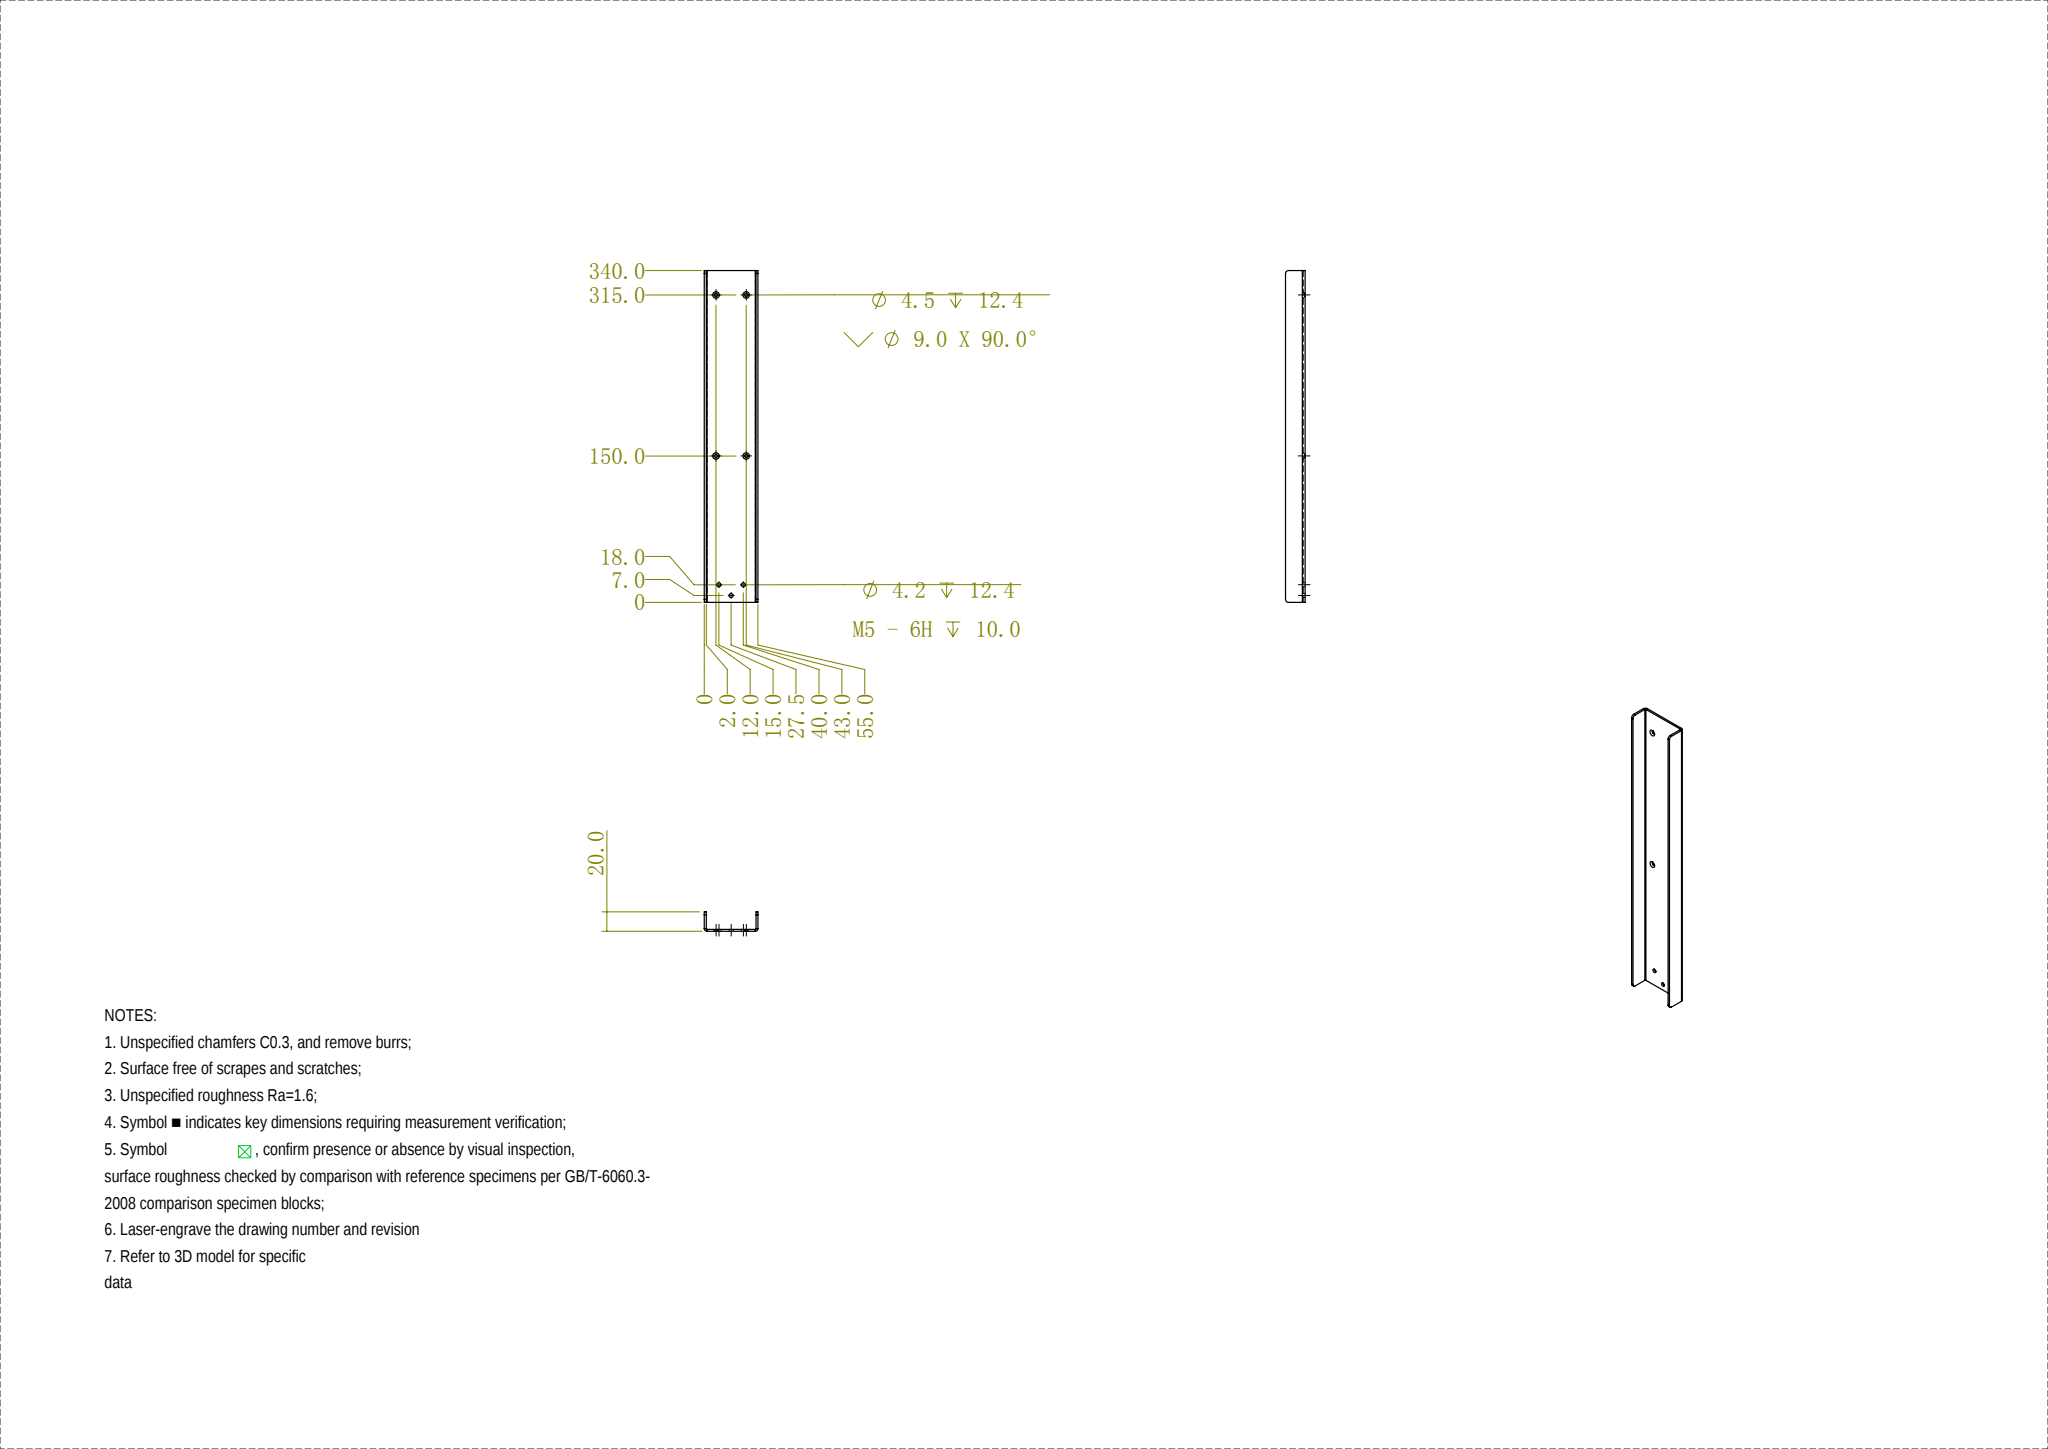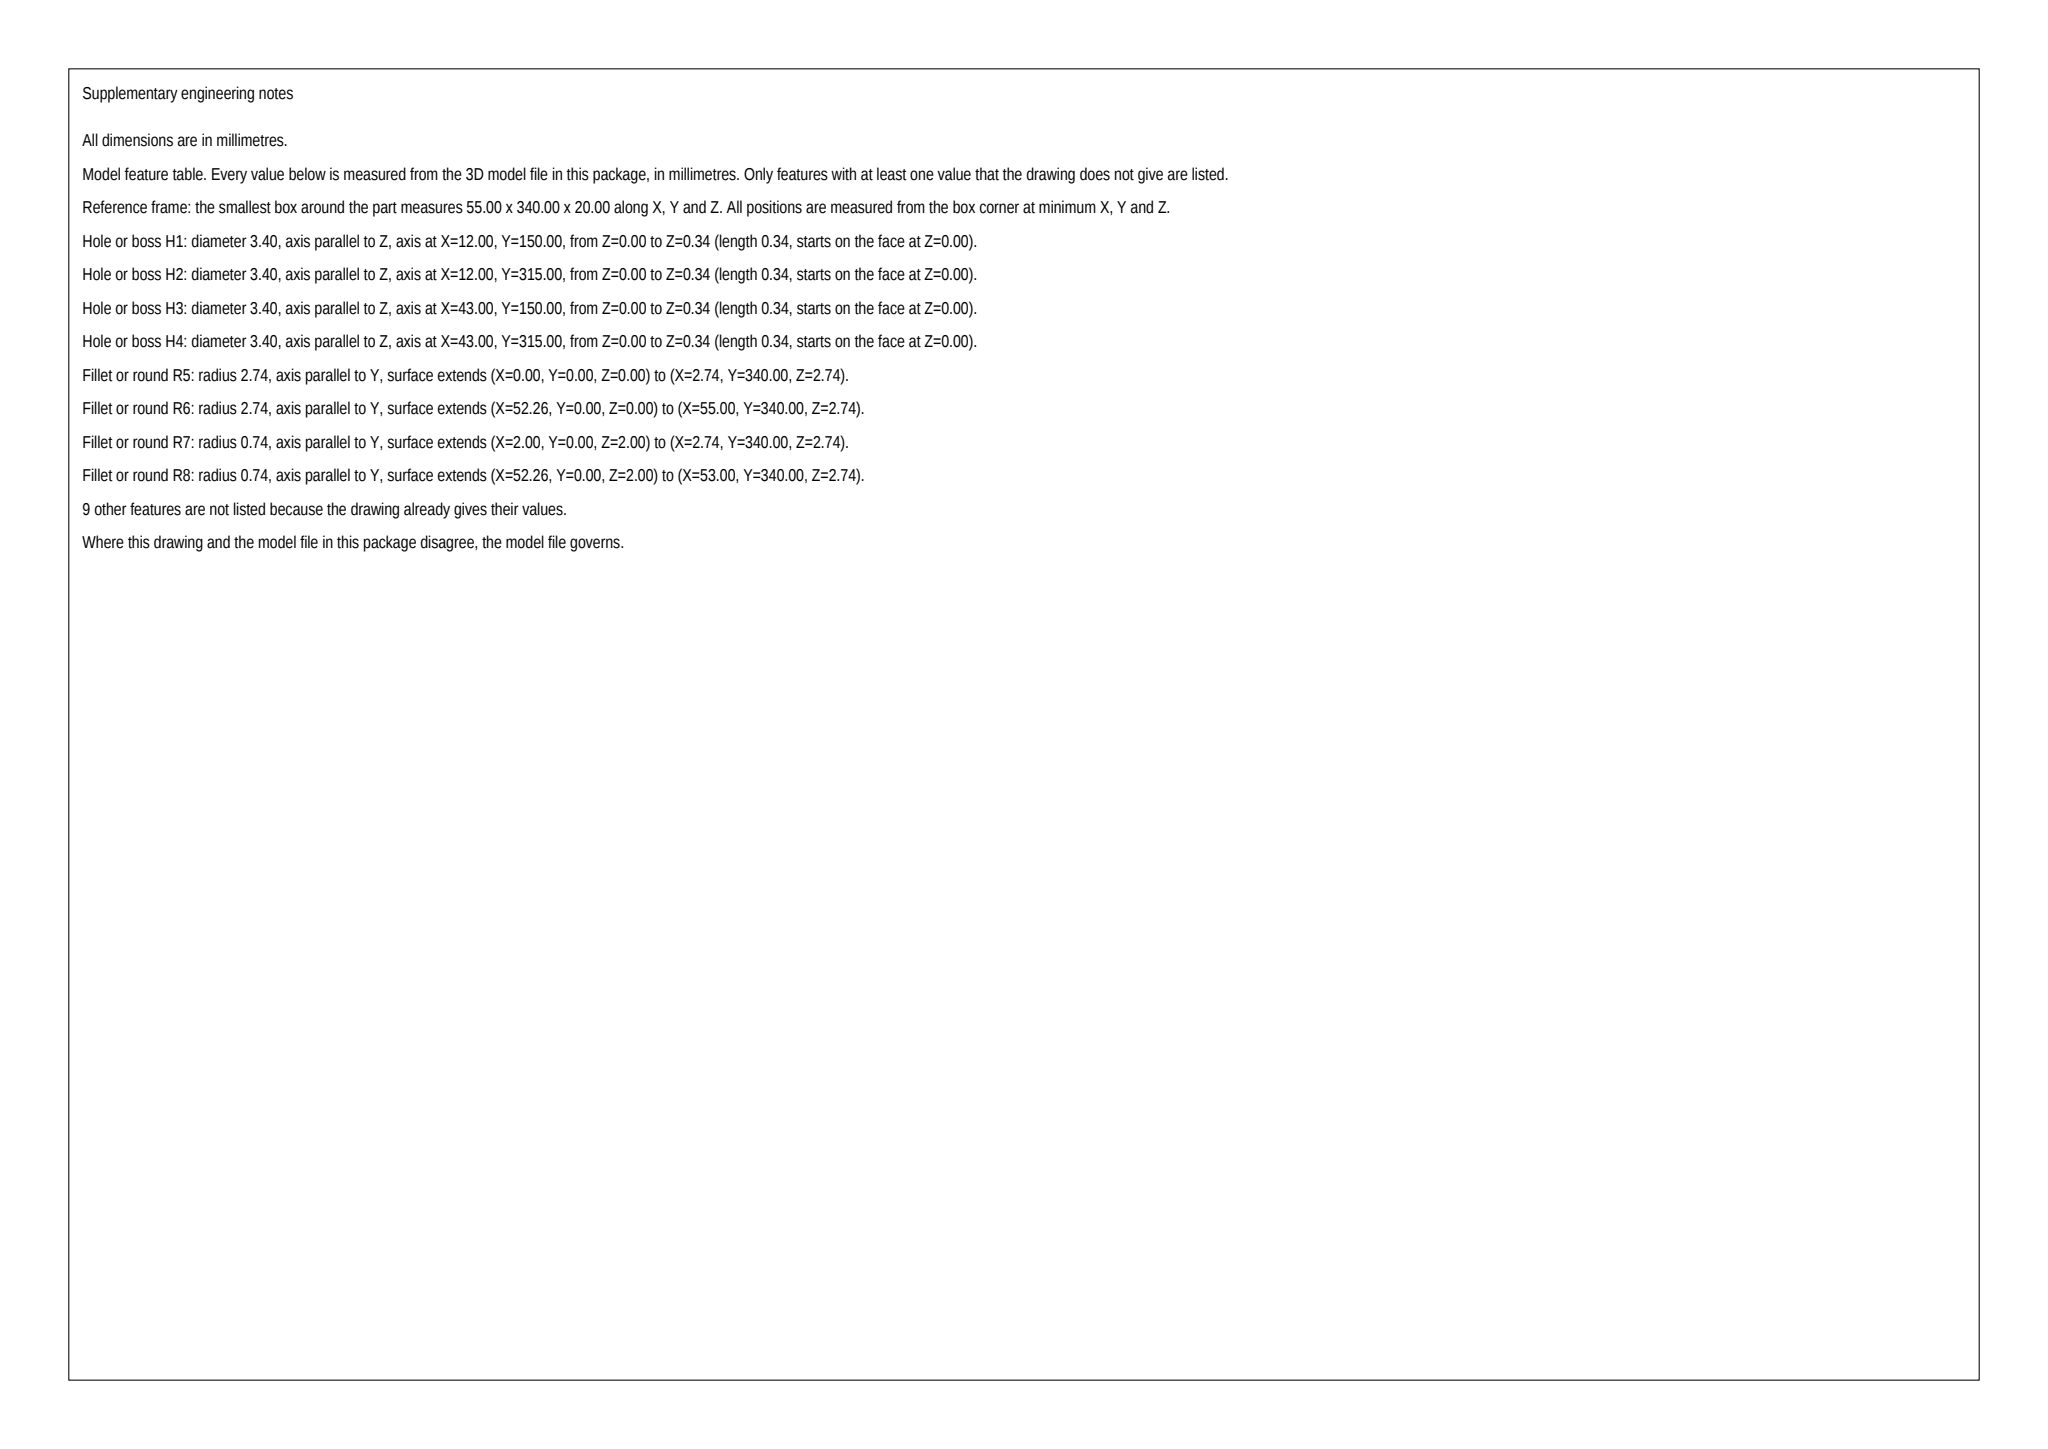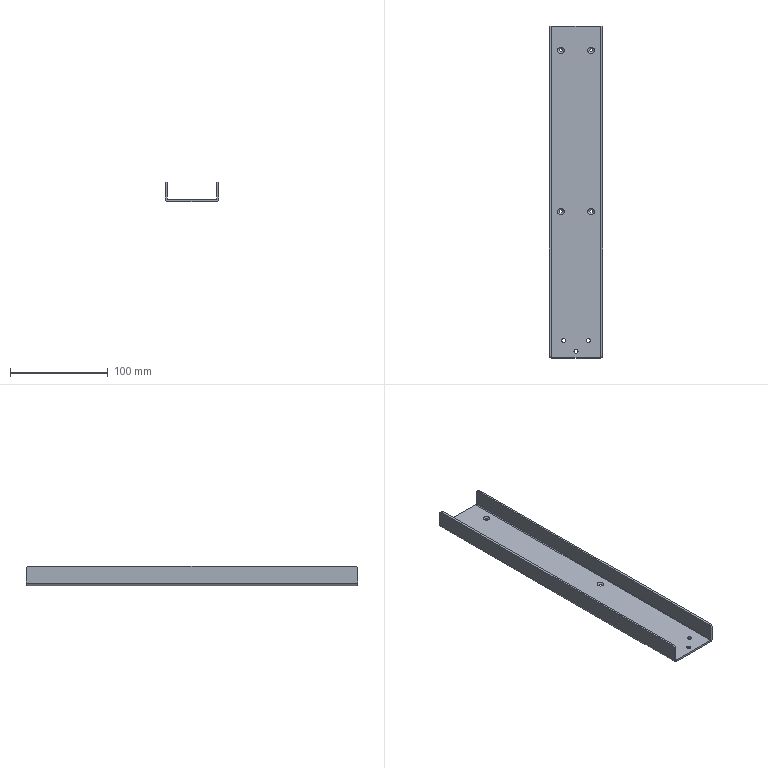Part | SolidWorks | mm | 1 solid | 48 faces | box 55 x 340 x 20 mm | volume 60617 mm3 | cylinder 22 | plane 18 | cone 8 | commonest cylinder face diameters 3.4 x8 4.2 x6 6 x4 5.473 x2 1.473 x2